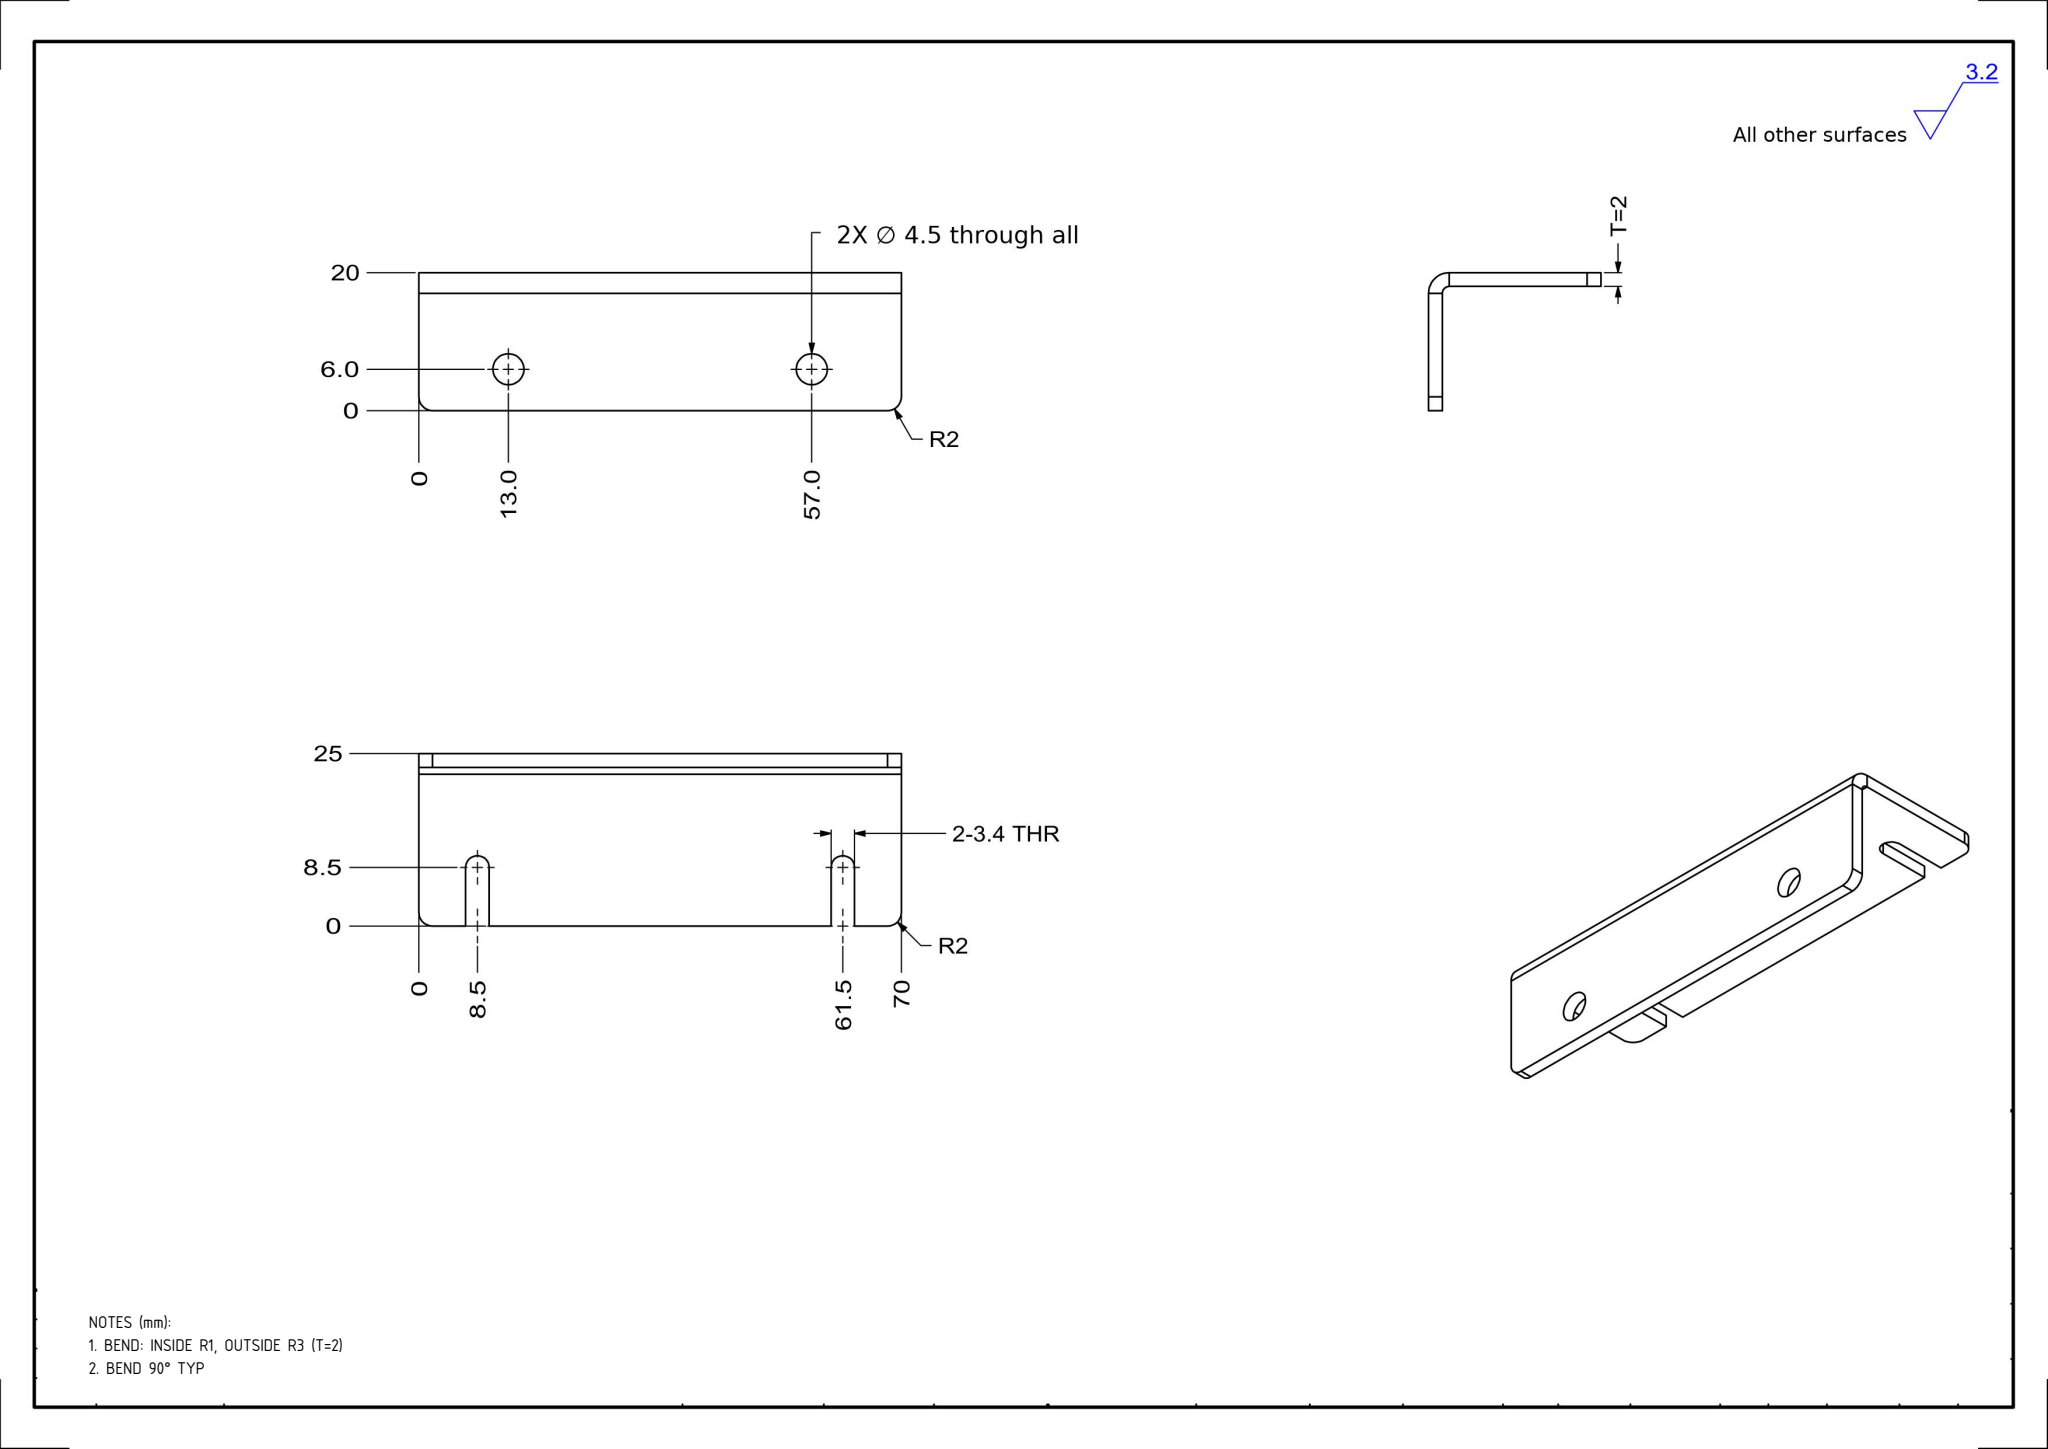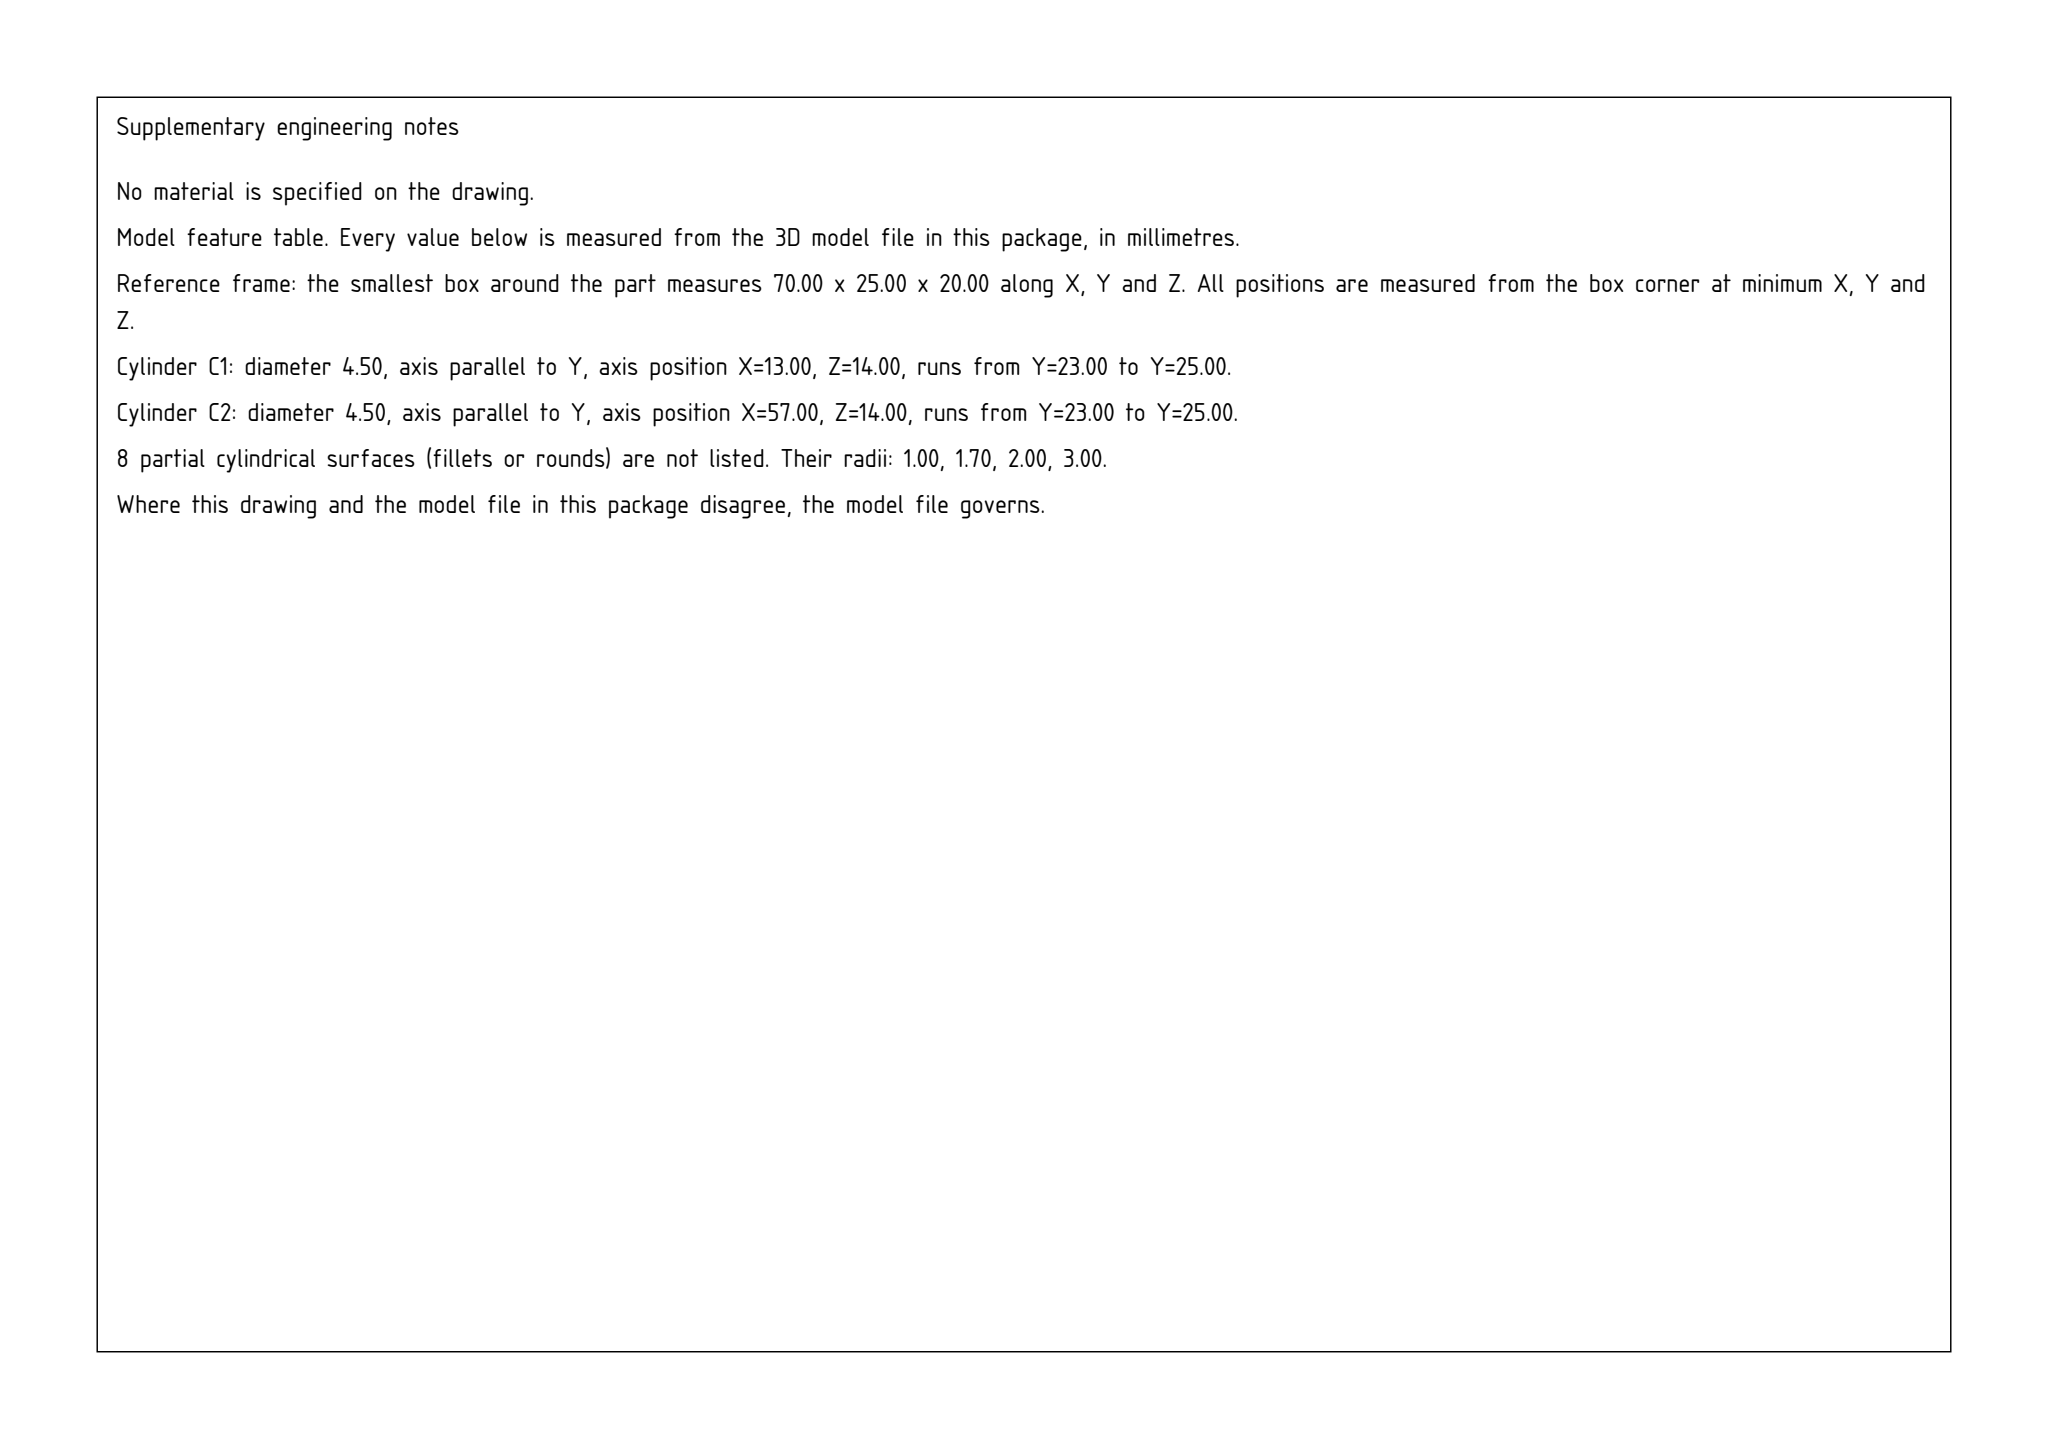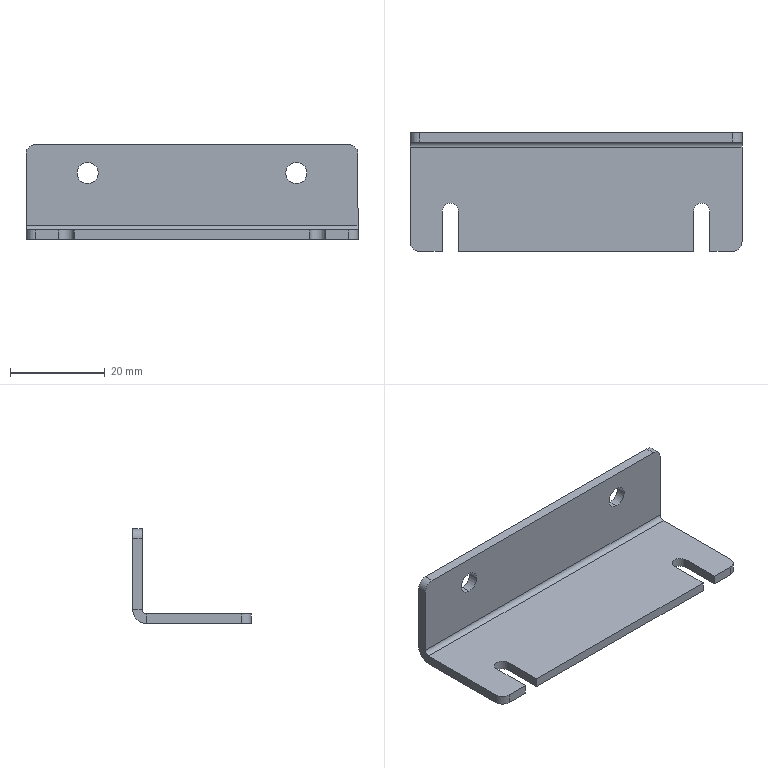Part | SolidWorks | mm | 1 solid | 30 faces | box 70 x 25 x 20 mm | volume 5696 mm3 | plane 18 | cylinder 12 | commonest cylinder face diameters 4.5 x4 4 x4 3.4 x2 6 x1 2 x1
Drawing notes:
BEND: INSIDE R1, OUTSIDE R3 (T=2) | from the solid: Ø2.0 x-axis cyl at (y22,z3) L70 = inner R1; Ø6.0 x-axis cyl same axis = outer R3; wall planes z0/z2 give T=2
BEND 90° TYP | from the solid: Planes z=0/z=2 (flange) normal to planes y=23/y=25 (web) meeting at bend axis x, i.e. 90° bend
STEP:
#1=CARTESIAN_POINT('',(22.,12.5,14.25));
#2=VERTEX_POINT('',#1);
#3=CARTESIAN_POINT('',(22.,12.5,9.75));
#4=VERTEX_POINT('',#3);
#5=CARTESIAN_POINT('',(22.,12.5,12.));
#6=DIRECTION('',(0.,-1.,0.));
#7=DIRECTION('',(0.,0.,-1.));
#8=AXIS2_PLACEMENT_3D('',#5,#6,#7);
#9=CIRCLE('',#8,2.25);
#10=EDGE_CURVE('',#2,#4,#9,.T.);
#11=ORIENTED_EDGE('',*,*,#10,.F.);
#12=CARTESIAN_POINT('',(22.,10.5,14.25));
#13=VERTEX_POINT('',#12);
#14=CARTESIAN_POINT('',(22.,10.5,14.25));
#15=DIRECTION('',(0.,-1.,0.));
#16=VECTOR('',#15,1000.);
#17=LINE('',#14,#16);
#18=EDGE_CURVE('',#2,#13,#17,.T.);
#19=ORIENTED_EDGE('',*,*,#18,.T.);
#20=CARTESIAN_POINT('',(22.,10.5,9.75));
#21=VERTEX_POINT('',#20);
#22=CARTESIAN_POINT('',(22.,10.5,12.));
#23=DIRECTION('',(0.,-1.,0.));
#24=DIRECTION('',(0.,0.,-1.));
#25=AXIS2_PLACEMENT_3D('',#22,#23,#24);
#26=CIRCLE('',#25,2.25);
#27=EDGE_CURVE('',#13,#21,#26,.T.);
#28=ORIENTED_EDGE('',*,*,#27,.T.);
#29=CARTESIAN_POINT('',(22.,10.5,9.75));
#30=DIRECTION('',(0.,-1.,0.));
#31=VECTOR('',#30,1000.);
#32=LINE('',#29,#31);
#33=EDGE_CURVE('',#4,#21,#32,.T.);
#34=ORIENTED_EDGE('',*,*,#33,.F.);
#35=EDGE_LOOP('',(#11,#19,#28,#34));
#36=FACE_OUTER_BOUND('',#35,.T.);
#37=CARTESIAN_POINT('',(22.,10.5,12.));
#38=DIRECTION('',(0.,-1.,0.));
#39=DIRECTION('',(0.,0.,-1.));
#40=AXIS2_PLACEMENT_3D('',#37,#38,#39);
#41=CYLINDRICAL_SURFACE('',#40,2.25);
#42=ADVANCED_FACE('',(#36),#41,.F.);
#43=CARTESIAN_POINT('',(-22.,12.5,14.25));
#44=VERTEX_POINT('',#43);
#45=CARTESIAN_POINT('',(-22.,12.5,9.75));
#46=VERTEX_POINT('',#45);
#47=CARTESIAN_POINT('',(-22.,12.5,12.));
#48=DIRECTION('',(0.,-1.,0.));
#49=DIRECTION('',(0.,0.,-1.));
#50=AXIS2_PLACEMENT_3D('',#47,#48,#49);
#51=CIRCLE('',#50,2.25);
#52=EDGE_CURVE('',#44,#46,#51,.T.);
#53=ORIENTED_EDGE('',*,*,#52,.F.);
#54=CARTESIAN_POINT('',(-22.,10.5,14.25));
#55=VERTEX_POINT('',#54);
#56=CARTESIAN_POINT('',(-22.,10.5,14.25));
#57=DIRECTION('',(0.,-1.,0.));
#58=VECTOR('',#57,1000.);
#59=LINE('',#56,#58);
#60=EDGE_CURVE('',#44,#55,#59,.T.);
#61=ORIENTED_EDGE('',*,*,#60,.T.);
#62=CARTESIAN_POINT('',(-22.,10.5,9.75));
#63=VERTEX_POINT('',#62);
#64=CARTESIAN_POINT('',(-22.,10.5,12.));
#65=DIRECTION('',(0.,-1.,0.));
#66=DIRECTION('',(0.,0.,-1.));
#67=AXIS2_PLACEMENT_3D('',#64,#65,#66);
#68=CIRCLE('',#67,2.25);
#69=EDGE_CURVE('',#55,#63,#68,.T.);
#70=ORIENTED_EDGE('',*,*,#69,.T.);
#71=CARTESIAN_POINT('',(-22.,10.5,9.75));
#72=DIRECTION('',(0.,-1.,0.));
#73=VECTOR('',#72,1000.);
#74=LINE('',#71,#73);
#75=EDGE_CURVE('',#46,#63,#74,.T.);
#76=ORIENTED_EDGE('',*,*,#75,.F.);
#77=EDGE_LOOP('',(#53,#61,#70,#76));
#78=FACE_OUTER_BOUND('',#77,.T.);
#79=CARTESIAN_POINT('',(-22.,10.5,12.));
#80=DIRECTION('',(0.,-1.,0.));
#81=DIRECTION('',(0.,0.,-1.));
#82=AXIS2_PLACEMENT_3D('',#79,#80,#81);
#83=CYLINDRICAL_SURFACE('',#82,2.25);
#84=ADVANCED_FACE('',(#78),#83,.F.);
#85=CARTESIAN_POINT('',(-33.,-12.5,0.));
#86=VERTEX_POINT('',#85);
#87=CARTESIAN_POINT('',(-28.2,-12.5,0.));
#88=VERTEX_POINT('',#87);
#89=CARTESIAN_POINT('',(-35.,-12.5,0.));
#90=DIRECTION('',(1.,0.,0.));
#91=VECTOR('',#90,1000.);
#92=LINE('',#89,#91);
#93=EDGE_CURVE('',#86,#88,#92,.T.);
#94=ORIENTED_EDGE('',*,*,#93,.F.);
#95=CARTESIAN_POINT('',(-33.,-12.5,-2.));
#96=VERTEX_POINT('',#95);
#97=CARTESIAN_POINT('',(-33.,-12.5,-2.));
#98=DIRECTION('',(0.,0.,-1.));
#99=VECTOR('',#98,1000.);
#100=LINE('',#97,#99);
#101=EDGE_CURVE('',#86,#96,#100,.T.);
#102=ORIENTED_EDGE('',*,*,#101,.T.);
#103=CARTESIAN_POINT('',(-28.2,-12.5,-2.));
#104=VERTEX_POINT('',#103);
#105=CARTESIAN_POINT('',(-35.,-12.5,-2.));
#106=DIRECTION('',(1.,0.,0.));
#107=VECTOR('',#106,1000.);
#108=LINE('',#105,#107);
#109=EDGE_CURVE('',#96,#104,#108,.T.);
#110=ORIENTED_EDGE('',*,*,#109,.T.);
#111=CARTESIAN_POINT('',(-28.2,-12.5,18.));
#112=DIRECTION('',(0.,0.,-1.));
#113=VECTOR('',#112,1000.);
#114=LINE('',#111,#113);
#115=EDGE_CURVE('',#88,#104,#114,.T.);
#116=ORIENTED_EDGE('',*,*,#115,.F.);
#117=EDGE_LOOP('',(#94,#102,#110,#116));
#118=FACE_OUTER_BOUND('',#117,.T.);
#119=CARTESIAN_POINT('',(-35.,-12.5,-2.));
#120=DIRECTION('',(0.,-1.,0.));
#121=DIRECTION('',(0.,0.,-1.));
#122=AXIS2_PLACEMENT_3D('',#119,#120,#121);
#123=PLANE('',#122);
#124=ADVANCED_FACE('',(#118),#123,.T.);
#125=CARTESIAN_POINT('',(-24.8,-12.5,0.));
#126=VERTEX_POINT('',#125);
#127=CARTESIAN_POINT('',(-24.8,-12.5,-2.));
#128=VERTEX_POINT('',#127);
#129=CARTESIAN_POINT('',(-24.8,-12.5,18.));
#130=DIRECTION('',(0.,0.,-1.));
#131=VECTOR('',#130,1000.);
#132=LINE('',#129,#131);
#133=EDGE_CURVE('',#126,#128,#132,.T.);
#134=ORIENTED_EDGE('',*,*,#133,.T.);
#135=CARTESIAN_POINT('',(24.8,-12.5,-2.));
#136=VERTEX_POINT('',#135);
#137=CARTESIAN_POINT('',(-35.,-12.5,-2.));
#138=DIRECTION('',(1.,0.,0.));
#139=VECTOR('',#138,1000.);
#140=LINE('',#137,#139);
#141=EDGE_CURVE('',#128,#136,#140,.T.);
#142=ORIENTED_EDGE('',*,*,#141,.T.);
#143=CARTESIAN_POINT('',(24.8,-12.5,0.));
#144=VERTEX_POINT('',#143);
#145=CARTESIAN_POINT('',(24.8,-12.5,18.));
#146=DIRECTION('',(0.,0.,-1.));
#147=VECTOR('',#146,1000.);
#148=LINE('',#145,#147);
#149=EDGE_CURVE('',#144,#136,#148,.T.);
#150=ORIENTED_EDGE('',*,*,#149,.F.);
#151=CARTESIAN_POINT('',(-35.,-12.5,0.));
#152=DIRECTION('',(1.,0.,0.));
#153=VECTOR('',#152,1000.);
#154=LINE('',#151,#153);
#155=EDGE_CURVE('',#126,#144,#154,.T.);
#156=ORIENTED_EDGE('',*,*,#155,.F.);
#157=EDGE_LOOP('',(#134,#142,#150,#156));
#158=FACE_OUTER_BOUND('',#157,.T.);
#159=CARTESIAN_POINT('',(-35.,-12.5,-2.));
#160=DIRECTION('',(0.,-1.,0.));
#161=DIRECTION('',(0.,0.,-1.));
#162=AXIS2_PLACEMENT_3D('',#159,#160,#161);
#163=PLANE('',#162);
#164=ADVANCED_FACE('',(#158),#163,.T.);
#165=CARTESIAN_POINT('',(-35.,9.5,-2.));
#166=VERTEX_POINT('',#165);
#167=CARTESIAN_POINT('',(-35.,-10.5,-2.));
#168=VERTEX_POINT('',#167);
#169=CARTESIAN_POINT('',(-35.,-12.5,-2.));
#170=DIRECTION('',(0.,-1.,0.));
#171=VECTOR('',#170,1000.);
#172=LINE('',#169,#171);
#173=EDGE_CURVE('',#166,#168,#172,.T.);
#174=ORIENTED_EDGE('',*,*,#173,.T.);
#175=CARTESIAN_POINT('',(-35.,-10.5,0.));
#176=VERTEX_POINT('',#175);
#177=CARTESIAN_POINT('',(-35.,-10.5,-2.));
#178=DIRECTION('',(0.,0.,1.));
#179=VECTOR('',#178,1000.);
#180=LINE('',#177,#179);
#181=EDGE_CURVE('',#168,#176,#180,.T.);
#182=ORIENTED_EDGE('',*,*,#181,.T.);
#183=CARTESIAN_POINT('',(-35.,9.5,-0.));
#184=VERTEX_POINT('',#183);
#185=CARTESIAN_POINT('',(-35.,-12.5,0.));
#186=DIRECTION('',(0.,-1.,0.));
#187=VECTOR('',#186,1000.);
#188=LINE('',#185,#187);
#189=EDGE_CURVE('',#184,#176,#188,.T.);
#190=ORIENTED_EDGE('',*,*,#189,.F.);
#191=CARTESIAN_POINT('',(-35.,9.5,-0.));
#192=DIRECTION('',(0.,0.,-1.));
#193=VECTOR('',#192,1000.);
#194=LINE('',#191,#193);
#195=EDGE_CURVE('',#184,#166,#194,.T.);
#196=ORIENTED_EDGE('',*,*,#195,.T.);
#197=EDGE_LOOP('',(#174,#182,#190,#196));
#198=FACE_OUTER_BOUND('',#197,.T.);
#199=CARTESIAN_POINT('',(-35.,-12.5,-2.));
#200=DIRECTION('',(-1.,0.,0.));
#201=DIRECTION('',(0.,0.,1.));
#202=AXIS2_PLACEMENT_3D('',#199,#200,#201);
#203=PLANE('',#202);
#204=ADVANCED_FACE('',(#198),#203,.T.);
#205=ORIENTED_EDGE('',*,*,#109,.F.);
#206=CARTESIAN_POINT('',(-33.,-10.5,-2.));
#207=DIRECTION('',(0.,0.,-1.));
#208=DIRECTION('',(-1.,0.,0.));
#209=AXIS2_PLACEMENT_3D('',#206,#207,#208);
#210=CIRCLE('',#209,2.);
#211=EDGE_CURVE('',#96,#168,#210,.T.);
#212=ORIENTED_EDGE('',*,*,#211,.T.);
#213=ORIENTED_EDGE('',*,*,#173,.F.);
#214=CARTESIAN_POINT('',(35.,9.5,-2.));
#215=VERTEX_POINT('',#214);
#216=CARTESIAN_POINT('',(-35.,9.5,-2.));
#217=DIRECTION('',(1.,0.,0.));
#218=VECTOR('',#217,1000.);
#219=LINE('',#216,#218);
#220=EDGE_CURVE('',#166,#215,#219,.T.);
#221=ORIENTED_EDGE('',*,*,#220,.T.);
#222=CARTESIAN_POINT('',(35.,-10.5,-2.));
#223=VERTEX_POINT('',#222);
#224=CARTESIAN_POINT('',(35.,-12.5,-2.));
#225=DIRECTION('',(0.,1.,0.));
#226=VECTOR('',#225,1000.);
#227=LINE('',#224,#226);
#228=EDGE_CURVE('',#223,#215,#227,.T.);
#229=ORIENTED_EDGE('',*,*,#228,.F.);
#230=CARTESIAN_POINT('',(33.,-12.5,-2.));
#231=VERTEX_POINT('',#230);
#232=CARTESIAN_POINT('',(33.,-10.5,-2.));
#233=DIRECTION('',(0.,0.,-1.));
#234=DIRECTION('',(-1.,0.,0.));
#235=AXIS2_PLACEMENT_3D('',#232,#233,#234);
#236=CIRCLE('',#235,2.);
#237=EDGE_CURVE('',#223,#231,#236,.T.);
#238=ORIENTED_EDGE('',*,*,#237,.T.);
#239=CARTESIAN_POINT('',(28.2,-12.5,-2.));
#240=VERTEX_POINT('',#239);
#241=CARTESIAN_POINT('',(-35.,-12.5,-2.));
#242=DIRECTION('',(1.,0.,0.));
#243=VECTOR('',#242,1000.);
#244=LINE('',#241,#243);
#245=EDGE_CURVE('',#240,#231,#244,.T.);
#246=ORIENTED_EDGE('',*,*,#245,.F.);
#247=CARTESIAN_POINT('',(28.2,-4.,-2.));
#248=VERTEX_POINT('',#247);
#249=CARTESIAN_POINT('',(28.2,-4.,-2.));
#250=DIRECTION('',(-0.,-1.,0.));
#251=VECTOR('',#250,1000.);
#252=LINE('',#249,#251);
#253=EDGE_CURVE('',#248,#240,#252,.T.);
#254=ORIENTED_EDGE('',*,*,#253,.F.);
#255=CARTESIAN_POINT('',(24.8,-4.,-2.));
#256=VERTEX_POINT('',#255);
#257=CARTESIAN_POINT('',(26.5,-4.,-2.));
#258=DIRECTION('',(0.,0.,-1.));
#259=DIRECTION('',(-1.,0.,0.));
#260=AXIS2_PLACEMENT_3D('',#257,#258,#259);
#261=CIRCLE('',#260,1.7);
#262=EDGE_CURVE('',#256,#248,#261,.T.);
#263=ORIENTED_EDGE('',*,*,#262,.F.);
#264=CARTESIAN_POINT('',(24.8,-4.,-2.));
#265=DIRECTION('',(0.,1.,0.));
#266=VECTOR('',#265,1000.);
#267=LINE('',#264,#266);
#268=EDGE_CURVE('',#136,#256,#267,.T.);
#269=ORIENTED_EDGE('',*,*,#268,.F.);
#270=ORIENTED_EDGE('',*,*,#141,.F.);
#271=CARTESIAN_POINT('',(-24.8,-4.,-2.));
#272=VERTEX_POINT('',#271);
#273=CARTESIAN_POINT('',(-24.8,-4.,-2.));
#274=DIRECTION('',(-0.,-1.,0.));
#275=VECTOR('',#274,1000.);
#276=LINE('',#273,#275);
#277=EDGE_CURVE('',#272,#128,#276,.T.);
#278=ORIENTED_EDGE('',*,*,#277,.F.);
#279=CARTESIAN_POINT('',(-28.2,-4.,-2.));
#280=VERTEX_POINT('',#279);
#281=CARTESIAN_POINT('',(-26.5,-4.,-2.));
#282=DIRECTION('',(0.,0.,-1.));
#283=DIRECTION('',(-1.,0.,0.));
#284=AXIS2_PLACEMENT_3D('',#281,#282,#283);
#285=CIRCLE('',#284,1.7);
#286=EDGE_CURVE('',#280,#272,#285,.T.);
#287=ORIENTED_EDGE('',*,*,#286,.F.);
#288=CARTESIAN_POINT('',(-28.2,-4.,-2.));
#289=DIRECTION('',(0.,1.,0.));
#290=VECTOR('',#289,1000.);
#291=LINE('',#288,#290);
#292=EDGE_CURVE('',#104,#280,#291,.T.);
#293=ORIENTED_EDGE('',*,*,#292,.F.);
#294=EDGE_LOOP('',(#205,#212,#213,#221,#229,#238,#246,#254,#263,#269,#270,#278,#287,#293));
#295=FACE_OUTER_BOUND('',#294,.T.);
#296=CARTESIAN_POINT('',(0.,0.,-2.));
#297=DIRECTION('',(0.,0.,-1.));
#298=DIRECTION('',(-1.,0.,0.));
#299=AXIS2_PLACEMENT_3D('',#296,#297,#298);
#300=PLANE('',#299);
#301=ADVANCED_FACE('',(#295),#300,.T.);
#302=ORIENTED_EDGE('',*,*,#189,.T.);
#303=CARTESIAN_POINT('',(-33.,-10.5,0.));
#304=DIRECTION('',(0.,0.,1.));
#305=DIRECTION('',(-1.,0.,0.));
#306=AXIS2_PLACEMENT_3D('',#303,#304,#305);
#307=CIRCLE('',#306,2.);
#308=EDGE_CURVE('',#176,#86,#307,.T.);
#309=ORIENTED_EDGE('',*,*,#308,.T.);
#310=ORIENTED_EDGE('',*,*,#93,.T.);
#311=CARTESIAN_POINT('',(-28.2,-4.,0.));
#312=VERTEX_POINT('',#311);
#313=CARTESIAN_POINT('',(-28.2,0.,0.));
#314=DIRECTION('',(0.,1.,0.));
#315=VECTOR('',#314,1000.);
#316=LINE('',#313,#315);
#317=EDGE_CURVE('',#88,#312,#316,.T.);
#318=ORIENTED_EDGE('',*,*,#317,.T.);
#319=CARTESIAN_POINT('',(-24.8,-4.,0.));
#320=VERTEX_POINT('',#319);
#321=CARTESIAN_POINT('',(-26.5,-4.,0.));
#322=DIRECTION('',(0.,0.,-1.));
#323=DIRECTION('',(-1.,0.,0.));
#324=AXIS2_PLACEMENT_3D('',#321,#322,#323);
#325=CIRCLE('',#324,1.7);
#326=EDGE_CURVE('',#312,#320,#325,.T.);
#327=ORIENTED_EDGE('',*,*,#326,.T.);
#328=CARTESIAN_POINT('',(-24.8,0.,0.));
#329=DIRECTION('',(-0.,-1.,0.));
#330=VECTOR('',#329,1000.);
#331=LINE('',#328,#330);
#332=EDGE_CURVE('',#320,#126,#331,.T.);
#333=ORIENTED_EDGE('',*,*,#332,.T.);
#334=ORIENTED_EDGE('',*,*,#155,.T.);
#335=CARTESIAN_POINT('',(24.8,-4.,0.));
#336=VERTEX_POINT('',#335);
#337=CARTESIAN_POINT('',(24.8,0.,0.));
#338=DIRECTION('',(0.,1.,0.));
#339=VECTOR('',#338,1000.);
#340=LINE('',#337,#339);
#341=EDGE_CURVE('',#144,#336,#340,.T.);
#342=ORIENTED_EDGE('',*,*,#341,.T.);
#343=CARTESIAN_POINT('',(28.2,-4.,0.));
#344=VERTEX_POINT('',#343);
#345=CARTESIAN_POINT('',(26.5,-4.,0.));
#346=DIRECTION('',(0.,0.,-1.));
#347=DIRECTION('',(-1.,0.,0.));
#348=AXIS2_PLACEMENT_3D('',#345,#346,#347);
#349=CIRCLE('',#348,1.7);
#350=EDGE_CURVE('',#336,#344,#349,.T.);
#351=ORIENTED_EDGE('',*,*,#350,.T.);
#352=CARTESIAN_POINT('',(28.2,-12.5,0.));
#353=VERTEX_POINT('',#352);
#354=CARTESIAN_POINT('',(28.2,-0.,0.));
#355=DIRECTION('',(-0.,-1.,0.));
#356=VECTOR('',#355,1000.);
#357=LINE('',#354,#356);
#358=EDGE_CURVE('',#344,#353,#357,.T.);
#359=ORIENTED_EDGE('',*,*,#358,.T.);
#360=CARTESIAN_POINT('',(33.,-12.5,0.));
#361=VERTEX_POINT('',#360);
#362=CARTESIAN_POINT('',(-35.,-12.5,0.));
#363=DIRECTION('',(1.,0.,0.));
#364=VECTOR('',#363,1000.);
#365=LINE('',#362,#364);
#366=EDGE_CURVE('',#353,#361,#365,.T.);
#367=ORIENTED_EDGE('',*,*,#366,.T.);
#368=CARTESIAN_POINT('',(35.,-10.5,0.));
#369=VERTEX_POINT('',#368);
#370=CARTESIAN_POINT('',(33.,-10.5,0.));
#371=DIRECTION('',(0.,0.,1.));
#372=DIRECTION('',(-1.,0.,0.));
#373=AXIS2_PLACEMENT_3D('',#370,#371,#372);
#374=CIRCLE('',#373,2.);
#375=EDGE_CURVE('',#361,#369,#374,.T.);
#376=ORIENTED_EDGE('',*,*,#375,.T.);
#377=CARTESIAN_POINT('',(35.,9.5,-0.));
#378=VERTEX_POINT('',#377);
#379=CARTESIAN_POINT('',(35.,-12.5,0.));
#380=DIRECTION('',(0.,1.,0.));
#381=VECTOR('',#380,1000.);
#382=LINE('',#379,#381);
#383=EDGE_CURVE('',#369,#378,#382,.T.);
#384=ORIENTED_EDGE('',*,*,#383,.T.);
#385=CARTESIAN_POINT('',(-35.,9.5,-0.));
#386=DIRECTION('',(1.,0.,0.));
#387=VECTOR('',#386,1000.);
#388=LINE('',#385,#387);
#389=EDGE_CURVE('',#184,#378,#388,.T.);
#390=ORIENTED_EDGE('',*,*,#389,.F.);
#391=EDGE_LOOP('',(#302,#309,#310,#318,#327,#333,#334,#342,#351,#359,#367,#376,#384,#390));
#392=FACE_OUTER_BOUND('',#391,.T.);
#393=CARTESIAN_POINT('',(0.,0.,0.));
#394=DIRECTION('',(0.,0.,-1.));
#395=DIRECTION('',(-1.,0.,0.));
#396=AXIS2_PLACEMENT_3D('',#393,#394,#395);
#397=PLANE('',#396);
#398=ADVANCED_FACE('',(#392),#397,.F.);
#399=ORIENTED_EDGE('',*,*,#383,.F.);
#400=CARTESIAN_POINT('',(35.,-10.5,-2.));
#401=DIRECTION('',(0.,0.,-1.));
#402=VECTOR('',#401,1000.);
#403=LINE('',#400,#402);
#404=EDGE_CURVE('',#369,#223,#403,.T.);
#405=ORIENTED_EDGE('',*,*,#404,.T.);
#406=ORIENTED_EDGE('',*,*,#228,.T.);
#407=CARTESIAN_POINT('',(35.,9.5,-0.));
#408=DIRECTION('',(0.,0.,-1.));
#409=VECTOR('',#408,1000.);
#410=LINE('',#407,#409);
#411=EDGE_CURVE('',#378,#215,#410,.T.);
#412=ORIENTED_EDGE('',*,*,#411,.F.);
#413=EDGE_LOOP('',(#399,#405,#406,#412));
#414=FACE_OUTER_BOUND('',#413,.T.);
#415=CARTESIAN_POINT('',(35.,-12.5,-2.));
#416=DIRECTION('',(1.,0.,0.));
#417=DIRECTION('',(0.,0.,-1.));
#418=AXIS2_PLACEMENT_3D('',#415,#416,#417);
#419=PLANE('',#418);
#420=ADVANCED_FACE('',(#414),#419,.T.);
#421=ORIENTED_EDGE('',*,*,#245,.T.);
#422=CARTESIAN_POINT('',(33.,-12.5,-2.));
#423=DIRECTION('',(0.,0.,1.));
#424=VECTOR('',#423,1000.);
#425=LINE('',#422,#424);
#426=EDGE_CURVE('',#231,#361,#425,.T.);
#427=ORIENTED_EDGE('',*,*,#426,.T.);
#428=ORIENTED_EDGE('',*,*,#366,.F.);
#429=CARTESIAN_POINT('',(28.2,-12.5,-2.));
#430=DIRECTION('',(0.,0.,1.));
#431=VECTOR('',#430,1000.);
#432=LINE('',#429,#431);
#433=EDGE_CURVE('',#240,#353,#432,.T.);
#434=ORIENTED_EDGE('',*,*,#433,.F.);
#435=EDGE_LOOP('',(#421,#427,#428,#434));
#436=FACE_OUTER_BOUND('',#435,.T.);
#437=CARTESIAN_POINT('',(-35.,-12.5,-2.));
#438=DIRECTION('',(0.,-1.,0.));
#439=DIRECTION('',(0.,0.,-1.));
#440=AXIS2_PLACEMENT_3D('',#437,#438,#439);
#441=PLANE('',#440);
#442=ADVANCED_FACE('',(#436),#441,.T.);
#443=CARTESIAN_POINT('',(35.,10.5,1.));
#444=VERTEX_POINT('',#443);
#445=CARTESIAN_POINT('',(35.,12.5,1.));
#446=VERTEX_POINT('',#445);
#447=CARTESIAN_POINT('',(35.,12.5,1.));
#448=DIRECTION('',(0.,1.,-0.));
#449=VECTOR('',#448,1000.);
#450=LINE('',#447,#449);
#451=EDGE_CURVE('',#444,#446,#450,.T.);
#452=ORIENTED_EDGE('',*,*,#451,.F.);
#453=CARTESIAN_POINT('',(35.,9.5,1.));
#454=DIRECTION('',(1.,0.,0.));
#455=DIRECTION('',(0.,0.,1.));
#456=AXIS2_PLACEMENT_3D('',#453,#454,#455);
#457=CIRCLE('',#456,1.);
#458=EDGE_CURVE('',#378,#444,#457,.T.);
#459=ORIENTED_EDGE('',*,*,#458,.F.);
#460=ORIENTED_EDGE('',*,*,#411,.T.);
#461=CARTESIAN_POINT('',(35.,9.5,1.));
#462=DIRECTION('',(1.,0.,0.));
#463=DIRECTION('',(0.,0.,1.));
#464=AXIS2_PLACEMENT_3D('',#461,#462,#463);
#465=CIRCLE('',#464,3.);
#466=EDGE_CURVE('',#215,#446,#465,.T.);
#467=ORIENTED_EDGE('',*,*,#466,.T.);
#468=EDGE_LOOP('',(#452,#459,#460,#467));
#469=FACE_OUTER_BOUND('',#468,.T.);
#470=CARTESIAN_POINT('',(35.,9.5,1.));
#471=DIRECTION('',(1.,0.,0.));
#472=DIRECTION('',(0.,0.,-1.));
#473=AXIS2_PLACEMENT_3D('',#470,#471,#472);
#474=PLANE('',#473);
#475=ADVANCED_FACE('',(#469),#474,.T.);
#476=CARTESIAN_POINT('',(-35.,10.5,1.));
#477=VERTEX_POINT('',#476);
#478=CARTESIAN_POINT('',(-35.,9.5,1.));
#479=DIRECTION('',(-1.,0.,0.));
#480=DIRECTION('',(0.,0.,1.));
#481=AXIS2_PLACEMENT_3D('',#478,#479,#480);
#482=CIRCLE('',#481,1.);
#483=EDGE_CURVE('',#477,#184,#482,.T.);
#484=ORIENTED_EDGE('',*,*,#483,.F.);
#485=CARTESIAN_POINT('',(-35.,12.5,1.));
#486=VERTEX_POINT('',#485);
#487=CARTESIAN_POINT('',(-35.,10.5,1.));
#488=DIRECTION('',(0.,1.,-0.));
#489=VECTOR('',#488,1000.);
#490=LINE('',#487,#489);
#491=EDGE_CURVE('',#477,#486,#490,.T.);
#492=ORIENTED_EDGE('',*,*,#491,.T.);
#493=CARTESIAN_POINT('',(-35.,9.5,1.));
#494=DIRECTION('',(-1.,0.,0.));
#495=DIRECTION('',(0.,0.,1.));
#496=AXIS2_PLACEMENT_3D('',#493,#494,#495);
#497=CIRCLE('',#496,3.);
#498=EDGE_CURVE('',#486,#166,#497,.T.);
#499=ORIENTED_EDGE('',*,*,#498,.T.);
#500=ORIENTED_EDGE('',*,*,#195,.F.);
#501=EDGE_LOOP('',(#484,#492,#499,#500));
#502=FACE_OUTER_BOUND('',#501,.T.);
#503=CARTESIAN_POINT('',(-35.,9.5,1.));
#504=DIRECTION('',(1.,0.,0.));
#505=DIRECTION('',(0.,0.,-1.));
#506=AXIS2_PLACEMENT_3D('',#503,#504,#505);
#507=PLANE('',#506);
#508=ADVANCED_FACE('',(#502),#507,.F.);
#509=ORIENTED_EDGE('',*,*,#220,.F.);
#510=ORIENTED_EDGE('',*,*,#498,.F.);
#511=CARTESIAN_POINT('',(35.,12.5,1.));
#512=DIRECTION('',(1.,0.,0.));
#513=VECTOR('',#512,1000.);
#514=LINE('',#511,#513);
#515=EDGE_CURVE('',#486,#446,#514,.T.);
#516=ORIENTED_EDGE('',*,*,#515,.T.);
#517=ORIENTED_EDGE('',*,*,#466,.F.);
#518=EDGE_LOOP('',(#509,#510,#516,#517));
#519=FACE_OUTER_BOUND('',#518,.T.);
#520=CARTESIAN_POINT('',(-35.,9.5,1.));
#521=DIRECTION('',(-1.,0.,0.));
#522=DIRECTION('',(0.,1.,-0.));
#523=AXIS2_PLACEMENT_3D('',#520,#521,#522);
#524=CYLINDRICAL_SURFACE('',#523,3.);
#525=ADVANCED_FACE('',(#519),#524,.T.);
#526=ORIENTED_EDGE('',*,*,#389,.T.);
#527=ORIENTED_EDGE('',*,*,#458,.T.);
#528=CARTESIAN_POINT('',(35.,10.5,1.));
#529=DIRECTION('',(-1.,0.,0.));
#530=VECTOR('',#529,1000.);
#531=LINE('',#528,#530);
#532=EDGE_CURVE('',#444,#477,#531,.T.);
#533=ORIENTED_EDGE('',*,*,#532,.T.);
#534=ORIENTED_EDGE('',*,*,#483,.T.);
#535=EDGE_LOOP('',(#526,#527,#533,#534));
#536=FACE_OUTER_BOUND('',#535,.T.);
#537=CARTESIAN_POINT('',(-35.,9.5,1.));
#538=DIRECTION('',(-1.,0.,0.));
#539=DIRECTION('',(0.,1.,-0.));
#540=AXIS2_PLACEMENT_3D('',#537,#538,#539);
#541=CYLINDRICAL_SURFACE('',#540,1.);
#542=ADVANCED_FACE('',(#536),#541,.F.);
#543=CARTESIAN_POINT('',(35.,12.5,16.));
#544=VERTEX_POINT('',#543);
#545=CARTESIAN_POINT('',(35.,12.5,0.));
#546=DIRECTION('',(0.,-0.,-1.));
#547=VECTOR('',#546,1000.);
#548=LINE('',#545,#547);
#549=EDGE_CURVE('',#544,#446,#548,.T.);
#550=ORIENTED_EDGE('',*,*,#549,.F.);
#551=CARTESIAN_POINT('',(35.,10.5,16.));
#552=VERTEX_POINT('',#551);
#553=CARTESIAN_POINT('',(35.,12.5,16.));
#554=DIRECTION('',(0.,-1.,0.));
#555=VECTOR('',#554,1000.);
#556=LINE('',#553,#555);
#557=EDGE_CURVE('',#544,#552,#556,.T.);
#558=ORIENTED_EDGE('',*,*,#557,.T.);
#559=CARTESIAN_POINT('',(35.,10.5,-0.));
#560=DIRECTION('',(0.,-0.,-1.));
#561=VECTOR('',#560,1000.);
#562=LINE('',#559,#561);
#563=EDGE_CURVE('',#552,#444,#562,.T.);
#564=ORIENTED_EDGE('',*,*,#563,.T.);
#565=ORIENTED_EDGE('',*,*,#451,.T.);
#566=EDGE_LOOP('',(#550,#558,#564,#565));
#567=FACE_OUTER_BOUND('',#566,.T.);
#568=CARTESIAN_POINT('',(35.,12.5,-0.));
#569=DIRECTION('',(-1.,-0.,-0.));
#570=DIRECTION('',(-0.,0.,1.));
#571=AXIS2_PLACEMENT_3D('',#568,#569,#570);
#572=PLANE('',#571);
#573=ADVANCED_FACE('',(#567),#572,.F.);
#574=CARTESIAN_POINT('',(-35.,10.5,16.));
#575=VERTEX_POINT('',#574);
#576=CARTESIAN_POINT('',(-35.,10.5,18.));
#577=DIRECTION('',(-0.,0.,1.));
#578=VECTOR('',#577,1000.);
#579=LINE('',#576,#578);
#580=EDGE_CURVE('',#477,#575,#579,.T.);
#581=ORIENTED_EDGE('',*,*,#580,.T.);
#582=CARTESIAN_POINT('',(-35.,12.5,16.));
#583=VERTEX_POINT('',#582);
#584=CARTESIAN_POINT('',(-35.,12.5,16.));
#585=DIRECTION('',(0.,1.,-0.));
#586=VECTOR('',#585,1000.);
#587=LINE('',#584,#586);
#588=EDGE_CURVE('',#575,#583,#587,.T.);
#589=ORIENTED_EDGE('',*,*,#588,.T.);
#590=CARTESIAN_POINT('',(-35.,12.5,-0.));
#591=DIRECTION('',(-0.,0.,1.));
#592=VECTOR('',#591,1000.);
#593=LINE('',#590,#592);
#594=EDGE_CURVE('',#486,#583,#593,.T.);
#595=ORIENTED_EDGE('',*,*,#594,.F.);
#596=ORIENTED_EDGE('',*,*,#491,.F.);
#597=EDGE_LOOP('',(#581,#589,#595,#596));
#598=FACE_OUTER_BOUND('',#597,.T.);
#599=CARTESIAN_POINT('',(-35.,12.5,18.));
#600=DIRECTION('',(1.,0.,0.));
#601=DIRECTION('',(0.,0.,-1.));
#602=AXIS2_PLACEMENT_3D('',#599,#600,#601);
#603=PLANE('',#602);
#604=ADVANCED_FACE('',(#598),#603,.F.);
#605=CARTESIAN_POINT('',(22.,12.5,12.));
#606=DIRECTION('',(0.,-1.,0.));
#607=DIRECTION('',(0.,0.,-1.));
#608=AXIS2_PLACEMENT_3D('',#605,#606,#607);
#609=CIRCLE('',#608,2.25);
#610=EDGE_CURVE('',#4,#2,#609,.T.);
#611=ORIENTED_EDGE('',*,*,#610,.T.);
#612=ORIENTED_EDGE('',*,*,#10,.T.);
#613=EDGE_LOOP('',(#611,#612));
#614=FACE_BOUND('',#613,.T.);
#615=CARTESIAN_POINT('',(-22.,12.5,12.));
#616=DIRECTION('',(0.,-1.,0.));
#617=DIRECTION('',(0.,0.,-1.));
#618=AXIS2_PLACEMENT_3D('',#615,#616,#617);
#619=CIRCLE('',#618,2.25);
#620=EDGE_CURVE('',#46,#44,#619,.T.);
#621=ORIENTED_EDGE('',*,*,#620,.T.);
#622=ORIENTED_EDGE('',*,*,#52,.T.);
#623=EDGE_LOOP('',(#621,#622));
#624=FACE_BOUND('',#623,.T.);
#625=ORIENTED_EDGE('',*,*,#594,.T.);
#626=CARTESIAN_POINT('',(-33.,12.5,18.));
#627=VERTEX_POINT('',#626);
#628=CARTESIAN_POINT('',(-33.,12.5,16.));
#629=DIRECTION('',(0.,1.,-0.));
#630=DIRECTION('',(0.,-0.,-1.));
#631=AXIS2_PLACEMENT_3D('',#628,#629,#630);
#632=CIRCLE('',#631,2.);
#633=EDGE_CURVE('',#583,#627,#632,.T.);
#634=ORIENTED_EDGE('',*,*,#633,.T.);
#635=CARTESIAN_POINT('',(33.,12.5,18.));
#636=VERTEX_POINT('',#635);
#637=CARTESIAN_POINT('',(0.,12.5,18.));
#638=DIRECTION('',(1.,0.,0.));
#639=VECTOR('',#638,1000.);
#640=LINE('',#637,#639);
#641=EDGE_CURVE('',#627,#636,#640,.T.);
#642=ORIENTED_EDGE('',*,*,#641,.T.);
#643=CARTESIAN_POINT('',(33.,12.5,16.));
#644=DIRECTION('',(0.,1.,-0.));
#645=DIRECTION('',(0.,-0.,-1.));
#646=AXIS2_PLACEMENT_3D('',#643,#644,#645);
#647=CIRCLE('',#646,2.);
#648=EDGE_CURVE('',#636,#544,#647,.T.);
#649=ORIENTED_EDGE('',*,*,#648,.T.);
#650=ORIENTED_EDGE('',*,*,#549,.T.);
#651=ORIENTED_EDGE('',*,*,#515,.F.);
#652=EDGE_LOOP('',(#625,#634,#642,#649,#650,#651));
#653=FACE_OUTER_BOUND('',#652,.T.);
#654=CARTESIAN_POINT('',(0.,12.5,-0.));
#655=DIRECTION('',(0.,-1.,0.));
#656=DIRECTION('',(0.,-0.,-1.));
#657=AXIS2_PLACEMENT_3D('',#654,#655,#656);
#658=PLANE('',#657);
#659=ADVANCED_FACE('',(#614,#624,#653),#658,.F.);
#660=CARTESIAN_POINT('',(22.,10.5,12.));
#661=DIRECTION('',(0.,-1.,0.));
#662=DIRECTION('',(0.,0.,-1.));
#663=AXIS2_PLACEMENT_3D('',#660,#661,#662);
#664=CIRCLE('',#663,2.25);
#665=EDGE_CURVE('',#21,#13,#664,.T.);
#666=ORIENTED_EDGE('',*,*,#665,.F.);
#667=ORIENTED_EDGE('',*,*,#27,.F.);
#668=EDGE_LOOP('',(#666,#667));
#669=FACE_BOUND('',#668,.T.);
#670=CARTESIAN_POINT('',(-22.,10.5,12.));
#671=DIRECTION('',(0.,-1.,0.));
#672=DIRECTION('',(0.,0.,-1.));
#673=AXIS2_PLACEMENT_3D('',#670,#671,#672);
#674=CIRCLE('',#673,2.25);
#675=EDGE_CURVE('',#63,#55,#674,.T.);
#676=ORIENTED_EDGE('',*,*,#675,.F.);
#677=ORIENTED_EDGE('',*,*,#69,.F.);
#678=EDGE_LOOP('',(#676,#677));
#679=FACE_BOUND('',#678,.T.);
#680=CARTESIAN_POINT('',(-33.,10.5,18.));
#681=VERTEX_POINT('',#680);
#682=CARTESIAN_POINT('',(33.,10.5,18.));
#683=VERTEX_POINT('',#682);
#684=CARTESIAN_POINT('',(35.,10.5,18.));
#685=DIRECTION('',(1.,0.,0.));
#686=VECTOR('',#685,1000.);
#687=LINE('',#684,#686);
#688=EDGE_CURVE('',#681,#683,#687,.T.);
#689=ORIENTED_EDGE('',*,*,#688,.F.);
#690=CARTESIAN_POINT('',(-33.,10.5,16.));
#691=DIRECTION('',(0.,-1.,0.));
#692=DIRECTION('',(0.,-0.,-1.));
#693=AXIS2_PLACEMENT_3D('',#690,#691,#692);
#694=CIRCLE('',#693,2.);
#695=EDGE_CURVE('',#681,#575,#694,.T.);
#696=ORIENTED_EDGE('',*,*,#695,.T.);
#697=ORIENTED_EDGE('',*,*,#580,.F.);
#698=ORIENTED_EDGE('',*,*,#532,.F.);
#699=ORIENTED_EDGE('',*,*,#563,.F.);
#700=CARTESIAN_POINT('',(33.,10.5,16.));
#701=DIRECTION('',(0.,-1.,0.));
#702=DIRECTION('',(0.,-0.,-1.));
#703=AXIS2_PLACEMENT_3D('',#700,#701,#702);
#704=CIRCLE('',#703,2.);
#705=EDGE_CURVE('',#552,#683,#704,.T.);
#706=ORIENTED_EDGE('',*,*,#705,.T.);
#707=EDGE_LOOP('',(#689,#696,#697,#698,#699,#706));
#708=FACE_OUTER_BOUND('',#707,.T.);
#709=CARTESIAN_POINT('',(0.,10.5,-0.));
#710=DIRECTION('',(0.,-1.,0.));
#711=DIRECTION('',(0.,-0.,-1.));
#712=AXIS2_PLACEMENT_3D('',#709,#710,#711);
#713=PLANE('',#712);
#714=ADVANCED_FACE('',(#669,#679,#708),#713,.T.);
#715=ORIENTED_EDGE('',*,*,#641,.F.);
#716=CARTESIAN_POINT('',(-33.,12.5,18.));
#717=DIRECTION('',(0.,-1.,0.));
#718=VECTOR('',#717,1000.);
#719=LINE('',#716,#718);
#720=EDGE_CURVE('',#627,#681,#719,.T.);
#721=ORIENTED_EDGE('',*,*,#720,.T.);
#722=ORIENTED_EDGE('',*,*,#688,.T.);
#723=CARTESIAN_POINT('',(33.,12.5,18.));
#724=DIRECTION('',(0.,1.,-0.));
#725=VECTOR('',#724,1000.);
#726=LINE('',#723,#725);
#727=EDGE_CURVE('',#683,#636,#726,.T.);
#728=ORIENTED_EDGE('',*,*,#727,.T.);
#729=EDGE_LOOP('',(#715,#721,#722,#728));
#730=FACE_OUTER_BOUND('',#729,.T.);
#731=CARTESIAN_POINT('',(35.,12.5,18.));
#732=DIRECTION('',(0.,-0.,-1.));
#733=DIRECTION('',(0.,1.,-0.));
#734=AXIS2_PLACEMENT_3D('',#731,#732,#733);
#735=PLANE('',#734);
#736=ADVANCED_FACE('',(#730),#735,.F.);
#737=CARTESIAN_POINT('',(24.8,-4.,18.));
#738=DIRECTION('',(0.,0.,-1.));
#739=VECTOR('',#738,1000.);
#740=LINE('',#737,#739);
#741=EDGE_CURVE('',#336,#256,#740,.T.);
#742=ORIENTED_EDGE('',*,*,#741,.T.);
#743=ORIENTED_EDGE('',*,*,#262,.T.);
#744=CARTESIAN_POINT('',(28.2,-4.,18.));
#745=DIRECTION('',(0.,0.,-1.));
#746=VECTOR('',#745,1000.);
#747=LINE('',#744,#746);
#748=EDGE_CURVE('',#344,#248,#747,.T.);
#749=ORIENTED_EDGE('',*,*,#748,.F.);
#750=ORIENTED_EDGE('',*,*,#350,.F.);
#751=EDGE_LOOP('',(#742,#743,#749,#750));
#752=FACE_OUTER_BOUND('',#751,.T.);
#753=CARTESIAN_POINT('',(26.5,-4.,18.));
#754=DIRECTION('',(0.,0.,-1.));
#755=DIRECTION('',(-1.,0.,0.));
#756=AXIS2_PLACEMENT_3D('',#753,#754,#755);
#757=CYLINDRICAL_SURFACE('',#756,1.7);
#758=ADVANCED_FACE('',(#752),#757,.F.);
#759=ORIENTED_EDGE('',*,*,#149,.T.);
#760=ORIENTED_EDGE('',*,*,#268,.T.);
#761=ORIENTED_EDGE('',*,*,#741,.F.);
#762=ORIENTED_EDGE('',*,*,#341,.F.);
#763=EDGE_LOOP('',(#759,#760,#761,#762));
#764=FACE_OUTER_BOUND('',#763,.T.);
#765=CARTESIAN_POINT('',(24.8,-4.,18.));
#766=DIRECTION('',(-1.,0.,0.));
#767=DIRECTION('',(0.,0.,1.));
#768=AXIS2_PLACEMENT_3D('',#765,#766,#767);
#769=PLANE('',#768);
#770=ADVANCED_FACE('',(#764),#769,.F.);
#771=ORIENTED_EDGE('',*,*,#748,.T.);
#772=ORIENTED_EDGE('',*,*,#253,.T.);
#773=ORIENTED_EDGE('',*,*,#433,.T.);
#774=ORIENTED_EDGE('',*,*,#358,.F.);
#775=EDGE_LOOP('',(#771,#772,#773,#774));
#776=FACE_OUTER_BOUND('',#775,.T.);
#777=CARTESIAN_POINT('',(28.2,-4.,18.));
#778=DIRECTION('',(1.,-0.,0.));
#779=DIRECTION('',(0.,1.,0.));
#780=AXIS2_PLACEMENT_3D('',#777,#778,#779);
#781=PLANE('',#780);
#782=ADVANCED_FACE('',(#776),#781,.F.);
#783=CARTESIAN_POINT('',(-28.2,-4.,18.));
#784=DIRECTION('',(0.,0.,-1.));
#785=VECTOR('',#784,1000.);
#786=LINE('',#783,#785);
#787=EDGE_CURVE('',#312,#280,#786,.T.);
#788=ORIENTED_EDGE('',*,*,#787,.T.);
#789=ORIENTED_EDGE('',*,*,#286,.T.);
#790=CARTESIAN_POINT('',(-24.8,-4.,18.));
#791=DIRECTION('',(0.,0.,-1.));
#792=VECTOR('',#791,1000.);
#793=LINE('',#790,#792);
#794=EDGE_CURVE('',#320,#272,#793,.T.);
#795=ORIENTED_EDGE('',*,*,#794,.F.);
#796=ORIENTED_EDGE('',*,*,#326,.F.);
#797=EDGE_LOOP('',(#788,#789,#795,#796));
#798=FACE_OUTER_BOUND('',#797,.T.);
#799=CARTESIAN_POINT('',(-26.5,-4.,18.));
#800=DIRECTION('',(0.,0.,-1.));
#801=DIRECTION('',(-1.,0.,0.));
#802=AXIS2_PLACEMENT_3D('',#799,#800,#801);
#803=CYLINDRICAL_SURFACE('',#802,1.7);
#804=ADVANCED_FACE('',(#798),#803,.F.);
#805=ORIENTED_EDGE('',*,*,#115,.T.);
#806=ORIENTED_EDGE('',*,*,#292,.T.);
#807=ORIENTED_EDGE('',*,*,#787,.F.);
#808=ORIENTED_EDGE('',*,*,#317,.F.);
#809=EDGE_LOOP('',(#805,#806,#807,#808));
#810=FACE_OUTER_BOUND('',#809,.T.);
#811=CARTESIAN_POINT('',(-28.2,-4.,18.));
#812=DIRECTION('',(-1.,0.,0.));
#813=DIRECTION('',(0.,0.,1.));
#814=AXIS2_PLACEMENT_3D('',#811,#812,#813);
#815=PLANE('',#814);
#816=ADVANCED_FACE('',(#810),#815,.F.);
#817=ORIENTED_EDGE('',*,*,#794,.T.);
#818=ORIENTED_EDGE('',*,*,#277,.T.);
#819=ORIENTED_EDGE('',*,*,#133,.F.);
#820=ORIENTED_EDGE('',*,*,#332,.F.);
#821=EDGE_LOOP('',(#817,#818,#819,#820));
#822=FACE_OUTER_BOUND('',#821,.T.);
#823=CARTESIAN_POINT('',(-24.8,-4.,18.));
#824=DIRECTION('',(1.,-0.,0.));
#825=DIRECTION('',(0.,1.,0.));
#826=AXIS2_PLACEMENT_3D('',#823,#824,#825);
#827=PLANE('',#826);
#828=ADVANCED_FACE('',(#822),#827,.F.);
#829=ORIENTED_EDGE('',*,*,#60,.F.);
#830=ORIENTED_EDGE('',*,*,#620,.F.);
#831=ORIENTED_EDGE('',*,*,#75,.T.);
#832=ORIENTED_EDGE('',*,*,#675,.T.);
#833=EDGE_LOOP('',(#829,#830,#831,#832));
#834=FACE_OUTER_BOUND('',#833,.T.);
#835=CARTESIAN_POINT('',(-22.,10.5,12.));
#836=DIRECTION('',(0.,-1.,0.));
#837=DIRECTION('',(0.,0.,-1.));
#838=AXIS2_PLACEMENT_3D('',#835,#836,#837);
#839=CYLINDRICAL_SURFACE('',#838,2.25);
#840=ADVANCED_FACE('',(#834),#839,.F.);
#841=ORIENTED_EDGE('',*,*,#18,.F.);
#842=ORIENTED_EDGE('',*,*,#610,.F.);
#843=ORIENTED_EDGE('',*,*,#33,.T.);
#844=ORIENTED_EDGE('',*,*,#665,.T.);
#845=EDGE_LOOP('',(#841,#842,#843,#844));
#846=FACE_OUTER_BOUND('',#845,.T.);
#847=CARTESIAN_POINT('',(22.,10.5,12.));
#848=DIRECTION('',(0.,-1.,0.));
#849=DIRECTION('',(0.,0.,-1.));
#850=AXIS2_PLACEMENT_3D('',#847,#848,#849);
#851=CYLINDRICAL_SURFACE('',#850,2.25);
#852=ADVANCED_FACE('',(#846),#851,.F.);
#853=ORIENTED_EDGE('',*,*,#633,.F.);
#854=ORIENTED_EDGE('',*,*,#588,.F.);
#855=ORIENTED_EDGE('',*,*,#695,.F.);
#856=ORIENTED_EDGE('',*,*,#720,.F.);
#857=EDGE_LOOP('',(#853,#854,#855,#856));
#858=FACE_OUTER_BOUND('',#857,.T.);
#859=CARTESIAN_POINT('',(-33.,12.5,16.));
#860=DIRECTION('',(0.,-1.,0.));
#861=DIRECTION('',(0.,-0.,-1.));
#862=AXIS2_PLACEMENT_3D('',#859,#860,#861);
#863=CYLINDRICAL_SURFACE('',#862,2.);
#864=ADVANCED_FACE('',(#858),#863,.T.);
#865=ORIENTED_EDGE('',*,*,#648,.F.);
#866=ORIENTED_EDGE('',*,*,#727,.F.);
#867=ORIENTED_EDGE('',*,*,#705,.F.);
#868=ORIENTED_EDGE('',*,*,#557,.F.);
#869=EDGE_LOOP('',(#865,#866,#867,#868));
#870=FACE_OUTER_BOUND('',#869,.T.);
#871=CARTESIAN_POINT('',(33.,12.5,16.));
#872=DIRECTION('',(0.,-1.,0.));
#873=DIRECTION('',(0.,-0.,-1.));
#874=AXIS2_PLACEMENT_3D('',#871,#872,#873);
#875=CYLINDRICAL_SURFACE('',#874,2.);
#876=ADVANCED_FACE('',(#870),#875,.T.);
#877=ORIENTED_EDGE('',*,*,#211,.F.);
#878=ORIENTED_EDGE('',*,*,#101,.F.);
#879=ORIENTED_EDGE('',*,*,#308,.F.);
#880=ORIENTED_EDGE('',*,*,#181,.F.);
#881=EDGE_LOOP('',(#877,#878,#879,#880));
#882=FACE_OUTER_BOUND('',#881,.T.);
#883=CARTESIAN_POINT('',(-33.,-10.5,-2.));
#884=DIRECTION('',(0.,0.,1.));
#885=DIRECTION('',(1.,0.,0.));
#886=AXIS2_PLACEMENT_3D('',#883,#884,#885);
#887=CYLINDRICAL_SURFACE('',#886,2.);
#888=ADVANCED_FACE('',(#882),#887,.T.);
#889=ORIENTED_EDGE('',*,*,#237,.F.);
#890=ORIENTED_EDGE('',*,*,#404,.F.);
#891=ORIENTED_EDGE('',*,*,#375,.F.);
#892=ORIENTED_EDGE('',*,*,#426,.F.);
#893=EDGE_LOOP('',(#889,#890,#891,#892));
#894=FACE_OUTER_BOUND('',#893,.T.);
#895=CARTESIAN_POINT('',(33.,-10.5,-2.));
#896=DIRECTION('',(0.,0.,1.));
#897=DIRECTION('',(1.,0.,0.));
#898=AXIS2_PLACEMENT_3D('',#895,#896,#897);
#899=CYLINDRICAL_SURFACE('',#898,2.);
#900=ADVANCED_FACE('',(#894),#899,.T.);
#901=CLOSED_SHELL('',(#42,#84,#124,#164,#204,#301,#398,#420,#442,#475,#508,#525,#542,#573,#604,#659,#714,#736,#758,#770,#782,#804,#816,#828,#840,#852,#864,#876,#888,#900));
#902=MANIFOLD_SOLID_BREP('',#901);
#903=CARTESIAN_POINT('',(0.,0.,0.));
#904=DIRECTION('',(0.,0.,1.));
#905=DIRECTION('',(1.,0.,0.));
#906=AXIS2_PLACEMENT_3D('',#903,#904,#905);
#907=(LENGTH_UNIT()NAMED_UNIT(*)SI_UNIT(.MILLI.,.METRE.));
#908=UNCERTAINTY_MEASURE_WITH_UNIT(LENGTH_MEASURE(0.00001),#907,'','');
#909=(NAMED_UNIT(*)PLANE_ANGLE_UNIT()SI_UNIT($,.RADIAN.));
#910=(NAMED_UNIT(*)SI_UNIT($,.STERADIAN.)SOLID_ANGLE_UNIT());
#911=(GEOMETRIC_REPRESENTATION_CONTEXT(3)GLOBAL_UNCERTAINTY_ASSIGNED_CONTEXT((#908))GLOBAL_UNIT_ASSIGNED_CONTEXT((#907,#909,#910))REPRESENTATION_CONTEXT('',''));
#912=ADVANCED_BREP_SHAPE_REPRESENTATION('',(#902,#906),#911);